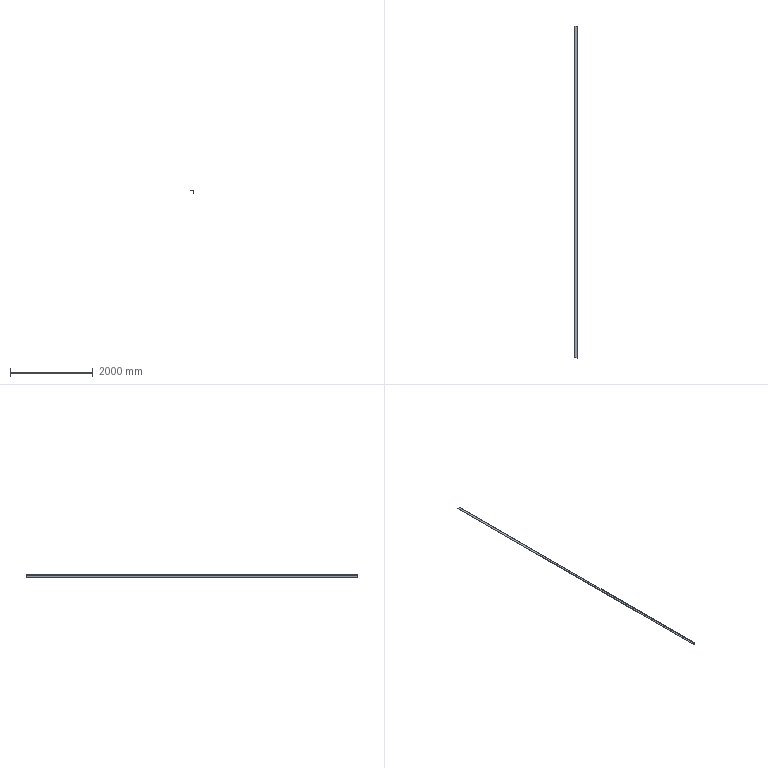Component | SolidWorks | 63#AngleIron-4 | 1 solid | 11 faces | box 63 x 8000 x 63 mm | volume 3982020 mm3 | plane 8 | cylinder 3 | commonest cylinder face diameters 2.667 x2 14 x1
build123d program:
from build123d import *

# Parameters (mm, degrees)
GB_T9787_1988_HOT_ROLLED_EQUAL_ANGLE_STE_DEPTH = 8000


with BuildPart() as part:
    # Sketch1 → Gb_t9787-1988 Hot Rolled Equal Angle Ste (new body)
    with BuildSketch(Plane.YZ):
        with BuildLine():
            Line((0, 0), (0, 63))
            Line((0, 63), (2.667, 63))
            ThreePointArc((2.667, 63), (3.609, 62.609), (4, 61.667))
            Line((4, 61.667), (4, 11))
            ThreePointArc((4, 11), (6.05, 6.05), (11, 4))
            Line((11, 4), (61.667, 4))
            ThreePointArc((61.667, 4), (62.609, 3.609), (63, 2.667))
            Line((63, 2.667), (63, 0))
            Line((63, 0), (0, 0))
        make_face()
    extrude(amount=GB_T9787_1988_HOT_ROLLED_EQUAL_ANGLE_STE_DEPTH)


solid = part.part

# Placed as in the assembly
solid = solid.moved(Location((2069.926, -31194.846, 4759), (-90, -90, 0)))
STEP:
#1=COLOUR_RGB('',0.7922,0.8196,0.9333);
#2=FILL_AREA_STYLE_COLOUR('',#1);
#3=FILL_AREA_STYLE('',(#2));
#4=SURFACE_STYLE_FILL_AREA(#3);
#5=SURFACE_SIDE_STYLE('',(#4));
#6=SURFACE_STYLE_USAGE(.BOTH.,#5);
#7=PRESENTATION_STYLE_ASSIGNMENT((#6));
#8=CARTESIAN_POINT('',(81.493,-1228.144,187.362));
#9=VERTEX_POINT('',#8);
#10=CARTESIAN_POINT('',(81.493,-1228.144,184.882));
#11=VERTEX_POINT('',#10);
#12=CARTESIAN_POINT('',(81.493,-1228.144,184.882));
#13=DIRECTION('',(-0.,-0.,-1.));
#14=VECTOR('',#13,39.37);
#15=LINE('',#12,#14);
#16=EDGE_CURVE('',#9,#11,#15,.T.);
#17=ORIENTED_EDGE('',*,*,#16,.T.);
#18=CARTESIAN_POINT('',(81.493,-913.183,184.882));
#19=VERTEX_POINT('',#18);
#20=CARTESIAN_POINT('',(81.493,-913.183,184.882));
#21=DIRECTION('',(-0.,-1.,0.));
#22=VECTOR('',#21,39.37);
#23=LINE('',#20,#22);
#24=EDGE_CURVE('',#19,#11,#23,.T.);
#25=ORIENTED_EDGE('',*,*,#24,.F.);
#26=CARTESIAN_POINT('',(81.493,-913.183,187.362));
#27=VERTEX_POINT('',#26);
#28=CARTESIAN_POINT('',(81.493,-913.183,184.882));
#29=DIRECTION('',(-0.,-0.,-1.));
#30=VECTOR('',#29,39.37);
#31=LINE('',#28,#30);
#32=EDGE_CURVE('',#27,#19,#31,.T.);
#33=ORIENTED_EDGE('',*,*,#32,.F.);
#34=CARTESIAN_POINT('',(81.493,-913.183,187.362));
#35=DIRECTION('',(-0.,-1.,0.));
#36=VECTOR('',#35,39.37);
#37=LINE('',#34,#36);
#38=EDGE_CURVE('',#27,#9,#37,.T.);
#39=ORIENTED_EDGE('',*,*,#38,.T.);
#40=EDGE_LOOP('',(#17,#25,#33,#39));
#41=FACE_OUTER_BOUND('',#40,.T.);
#42=CARTESIAN_POINT('',(81.493,-913.183,184.882));
#43=DIRECTION('',(-1.,0.,0.));
#44=DIRECTION('',(0.,1.,-0.));
#45=AXIS2_PLACEMENT_3D('',#42,#43,#44);
#46=PLANE('',#45);
#47=ADVANCED_FACE('',(#41),#46,.F.);
#48=CARTESIAN_POINT('',(81.388,-1228.144,184.882));
#49=VERTEX_POINT('',#48);
#50=CARTESIAN_POINT('',(81.493,-1228.144,184.882));
#51=DIRECTION('',(-1.,0.,0.));
#52=VECTOR('',#51,39.37);
#53=LINE('',#50,#52);
#54=EDGE_CURVE('',#11,#49,#53,.T.);
#55=ORIENTED_EDGE('',*,*,#54,.T.);
#56=CARTESIAN_POINT('',(81.388,-913.183,184.882));
#57=VERTEX_POINT('',#56);
#58=CARTESIAN_POINT('',(81.388,-913.183,184.882));
#59=DIRECTION('',(-0.,-1.,0.));
#60=VECTOR('',#59,39.37);
#61=LINE('',#58,#60);
#62=EDGE_CURVE('',#57,#49,#61,.T.);
#63=ORIENTED_EDGE('',*,*,#62,.F.);
#64=CARTESIAN_POINT('',(81.493,-913.183,184.882));
#65=DIRECTION('',(-1.,0.,0.));
#66=VECTOR('',#65,39.37);
#67=LINE('',#64,#66);
#68=EDGE_CURVE('',#19,#57,#67,.T.);
#69=ORIENTED_EDGE('',*,*,#68,.F.);
#70=ORIENTED_EDGE('',*,*,#24,.T.);
#71=EDGE_LOOP('',(#55,#63,#69,#70));
#72=FACE_OUTER_BOUND('',#71,.T.);
#73=CARTESIAN_POINT('',(81.493,-913.183,184.882));
#74=DIRECTION('',(0.,0.,1.));
#75=DIRECTION('',(1.,-0.,-0.));
#76=AXIS2_PLACEMENT_3D('',#73,#74,#75);
#77=PLANE('',#76);
#78=ADVANCED_FACE('',(#72),#77,.F.);
#79=CARTESIAN_POINT('',(81.336,-1228.144,184.934));
#80=VERTEX_POINT('',#79);
#81=CARTESIAN_POINT('',(81.388,-1228.144,184.934));
#82=DIRECTION('',(0.,1.,-0.));
#83=DIRECTION('',(1.,0.,0.));
#84=AXIS2_PLACEMENT_3D('',#81,#82,#83);
#85=CIRCLE('',#84,0.05249);
#86=EDGE_CURVE('',#49,#80,#85,.T.);
#87=ORIENTED_EDGE('',*,*,#86,.T.);
#88=CARTESIAN_POINT('',(81.336,-913.183,184.934));
#89=VERTEX_POINT('',#88);
#90=CARTESIAN_POINT('',(81.336,-913.183,184.934));
#91=DIRECTION('',(-0.,-1.,0.));
#92=VECTOR('',#91,39.37);
#93=LINE('',#90,#92);
#94=EDGE_CURVE('',#89,#80,#93,.T.);
#95=ORIENTED_EDGE('',*,*,#94,.F.);
#96=CARTESIAN_POINT('',(81.388,-913.183,184.934));
#97=DIRECTION('',(0.,1.,-0.));
#98=DIRECTION('',(1.,0.,0.));
#99=AXIS2_PLACEMENT_3D('',#96,#97,#98);
#100=CIRCLE('',#99,0.05249);
#101=EDGE_CURVE('',#57,#89,#100,.T.);
#102=ORIENTED_EDGE('',*,*,#101,.F.);
#103=ORIENTED_EDGE('',*,*,#62,.T.);
#104=EDGE_LOOP('',(#87,#95,#102,#103));
#105=FACE_OUTER_BOUND('',#104,.T.);
#106=CARTESIAN_POINT('',(81.388,-913.183,184.934));
#107=DIRECTION('',(-0.,-1.,0.));
#108=DIRECTION('',(-1.,0.,0.));
#109=AXIS2_PLACEMENT_3D('',#106,#107,#108);
#110=CYLINDRICAL_SURFACE('',#109,0.05249);
#111=ADVANCED_FACE('',(#105),#110,.T.);
#112=CARTESIAN_POINT('',(81.336,-1228.144,186.929));
#113=VERTEX_POINT('',#112);
#114=CARTESIAN_POINT('',(81.336,-1228.144,186.929));
#115=DIRECTION('',(0.,0.,1.));
#116=VECTOR('',#115,39.37);
#117=LINE('',#114,#116);
#118=EDGE_CURVE('',#80,#113,#117,.T.);
#119=ORIENTED_EDGE('',*,*,#118,.T.);
#120=CARTESIAN_POINT('',(81.336,-913.183,186.929));
#121=VERTEX_POINT('',#120);
#122=CARTESIAN_POINT('',(81.336,-913.183,186.929));
#123=DIRECTION('',(-0.,-1.,0.));
#124=VECTOR('',#123,39.37);
#125=LINE('',#122,#124);
#126=EDGE_CURVE('',#121,#113,#125,.T.);
#127=ORIENTED_EDGE('',*,*,#126,.F.);
#128=CARTESIAN_POINT('',(81.336,-913.183,186.929));
#129=DIRECTION('',(0.,0.,1.));
#130=VECTOR('',#129,39.37);
#131=LINE('',#128,#130);
#132=EDGE_CURVE('',#89,#121,#131,.T.);
#133=ORIENTED_EDGE('',*,*,#132,.F.);
#134=ORIENTED_EDGE('',*,*,#94,.T.);
#135=EDGE_LOOP('',(#119,#127,#133,#134));
#136=FACE_OUTER_BOUND('',#135,.T.);
#137=CARTESIAN_POINT('',(81.336,-913.183,186.929));
#138=DIRECTION('',(1.,-0.,-0.));
#139=DIRECTION('',(-0.,-0.,-1.));
#140=AXIS2_PLACEMENT_3D('',#137,#138,#139);
#141=PLANE('',#140);
#142=ADVANCED_FACE('',(#136),#141,.F.);
#143=CARTESIAN_POINT('',(81.06,-1228.144,187.205));
#144=VERTEX_POINT('',#143);
#145=CARTESIAN_POINT('',(81.06,-1228.144,186.929));
#146=DIRECTION('',(-0.,-1.,0.));
#147=DIRECTION('',(-1.,0.,0.));
#148=AXIS2_PLACEMENT_3D('',#145,#146,#147);
#149=CIRCLE('',#148,0.2756);
#150=EDGE_CURVE('',#113,#144,#149,.T.);
#151=ORIENTED_EDGE('',*,*,#150,.T.);
#152=CARTESIAN_POINT('',(81.06,-913.183,187.205));
#153=VERTEX_POINT('',#152);
#154=CARTESIAN_POINT('',(81.06,-913.183,187.205));
#155=DIRECTION('',(-0.,-1.,0.));
#156=VECTOR('',#155,39.37);
#157=LINE('',#154,#156);
#158=EDGE_CURVE('',#153,#144,#157,.T.);
#159=ORIENTED_EDGE('',*,*,#158,.F.);
#160=CARTESIAN_POINT('',(81.06,-913.183,186.929));
#161=DIRECTION('',(-0.,-1.,0.));
#162=DIRECTION('',(-1.,0.,0.));
#163=AXIS2_PLACEMENT_3D('',#160,#161,#162);
#164=CIRCLE('',#163,0.2756);
#165=EDGE_CURVE('',#121,#153,#164,.T.);
#166=ORIENTED_EDGE('',*,*,#165,.F.);
#167=ORIENTED_EDGE('',*,*,#126,.T.);
#168=EDGE_LOOP('',(#151,#159,#166,#167));
#169=FACE_OUTER_BOUND('',#168,.T.);
#170=CARTESIAN_POINT('',(81.06,-913.183,186.929));
#171=DIRECTION('',(-0.,-1.,0.));
#172=DIRECTION('',(-1.,0.,0.));
#173=AXIS2_PLACEMENT_3D('',#170,#171,#172);
#174=CYLINDRICAL_SURFACE('',#173,0.2756);
#175=ADVANCED_FACE('',(#169),#174,.F.);
#176=CARTESIAN_POINT('',(79.065,-1228.144,187.205));
#177=VERTEX_POINT('',#176);
#178=CARTESIAN_POINT('',(79.065,-1228.144,187.205));
#179=DIRECTION('',(-1.,0.,0.));
#180=VECTOR('',#179,39.37);
#181=LINE('',#178,#180);
#182=EDGE_CURVE('',#144,#177,#181,.T.);
#183=ORIENTED_EDGE('',*,*,#182,.T.);
#184=CARTESIAN_POINT('',(79.065,-913.183,187.205));
#185=VERTEX_POINT('',#184);
#186=CARTESIAN_POINT('',(79.065,-913.183,187.205));
#187=DIRECTION('',(-0.,-1.,0.));
#188=VECTOR('',#187,39.37);
#189=LINE('',#186,#188);
#190=EDGE_CURVE('',#185,#177,#189,.T.);
#191=ORIENTED_EDGE('',*,*,#190,.F.);
#192=CARTESIAN_POINT('',(79.065,-913.183,187.205));
#193=DIRECTION('',(-1.,0.,0.));
#194=VECTOR('',#193,39.37);
#195=LINE('',#192,#194);
#196=EDGE_CURVE('',#153,#185,#195,.T.);
#197=ORIENTED_EDGE('',*,*,#196,.F.);
#198=ORIENTED_EDGE('',*,*,#158,.T.);
#199=EDGE_LOOP('',(#183,#191,#197,#198));
#200=FACE_OUTER_BOUND('',#199,.T.);
#201=CARTESIAN_POINT('',(79.065,-913.183,187.205));
#202=DIRECTION('',(0.,0.,1.));
#203=DIRECTION('',(1.,-0.,-0.));
#204=AXIS2_PLACEMENT_3D('',#201,#202,#203);
#205=PLANE('',#204);
#206=ADVANCED_FACE('',(#200),#205,.F.);
#207=CARTESIAN_POINT('',(79.013,-1228.144,187.257));
#208=VERTEX_POINT('',#207);
#209=CARTESIAN_POINT('',(79.065,-1228.144,187.257));
#210=DIRECTION('',(0.,1.,-0.));
#211=DIRECTION('',(-1.,0.,0.));
#212=AXIS2_PLACEMENT_3D('',#209,#210,#211);
#213=CIRCLE('',#212,0.05249);
#214=EDGE_CURVE('',#177,#208,#213,.T.);
#215=ORIENTED_EDGE('',*,*,#214,.T.);
#216=CARTESIAN_POINT('',(79.013,-913.183,187.257));
#217=VERTEX_POINT('',#216);
#218=CARTESIAN_POINT('',(79.013,-913.183,187.257));
#219=DIRECTION('',(-0.,-1.,0.));
#220=VECTOR('',#219,39.37);
#221=LINE('',#218,#220);
#222=EDGE_CURVE('',#217,#208,#221,.T.);
#223=ORIENTED_EDGE('',*,*,#222,.F.);
#224=CARTESIAN_POINT('',(79.065,-913.183,187.257));
#225=DIRECTION('',(0.,1.,-0.));
#226=DIRECTION('',(-1.,0.,0.));
#227=AXIS2_PLACEMENT_3D('',#224,#225,#226);
#228=CIRCLE('',#227,0.05249);
#229=EDGE_CURVE('',#185,#217,#228,.T.);
#230=ORIENTED_EDGE('',*,*,#229,.F.);
#231=ORIENTED_EDGE('',*,*,#190,.T.);
#232=EDGE_LOOP('',(#215,#223,#230,#231));
#233=FACE_OUTER_BOUND('',#232,.T.);
#234=CARTESIAN_POINT('',(79.065,-913.183,187.257));
#235=DIRECTION('',(-0.,-1.,0.));
#236=DIRECTION('',(-1.,0.,0.));
#237=AXIS2_PLACEMENT_3D('',#234,#235,#236);
#238=CYLINDRICAL_SURFACE('',#237,0.05249);
#239=ADVANCED_FACE('',(#233),#238,.T.);
#240=CARTESIAN_POINT('',(79.013,-1228.144,187.362));
#241=VERTEX_POINT('',#240);
#242=CARTESIAN_POINT('',(79.013,-1228.144,187.362));
#243=DIRECTION('',(0.,0.,1.));
#244=VECTOR('',#243,39.37);
#245=LINE('',#242,#244);
#246=EDGE_CURVE('',#208,#241,#245,.T.);
#247=ORIENTED_EDGE('',*,*,#246,.T.);
#248=CARTESIAN_POINT('',(79.013,-913.183,187.362));
#249=VERTEX_POINT('',#248);
#250=CARTESIAN_POINT('',(79.013,-913.183,187.362));
#251=DIRECTION('',(-0.,-1.,0.));
#252=VECTOR('',#251,39.37);
#253=LINE('',#250,#252);
#254=EDGE_CURVE('',#249,#241,#253,.T.);
#255=ORIENTED_EDGE('',*,*,#254,.F.);
#256=CARTESIAN_POINT('',(79.013,-913.183,187.362));
#257=DIRECTION('',(0.,0.,1.));
#258=VECTOR('',#257,39.37);
#259=LINE('',#256,#258);
#260=EDGE_CURVE('',#217,#249,#259,.T.);
#261=ORIENTED_EDGE('',*,*,#260,.F.);
#262=ORIENTED_EDGE('',*,*,#222,.T.);
#263=EDGE_LOOP('',(#247,#255,#261,#262));
#264=FACE_OUTER_BOUND('',#263,.T.);
#265=CARTESIAN_POINT('',(79.013,-913.183,187.362));
#266=DIRECTION('',(1.,-0.,-0.));
#267=DIRECTION('',(-0.,-1.,0.));
#268=AXIS2_PLACEMENT_3D('',#265,#266,#267);
#269=PLANE('',#268);
#270=ADVANCED_FACE('',(#264),#269,.F.);
#271=CARTESIAN_POINT('',(81.493,-1228.144,187.362));
#272=DIRECTION('',(1.,-0.,-0.));
#273=VECTOR('',#272,39.37);
#274=LINE('',#271,#273);
#275=EDGE_CURVE('',#241,#9,#274,.T.);
#276=ORIENTED_EDGE('',*,*,#275,.T.);
#277=ORIENTED_EDGE('',*,*,#38,.F.);
#278=CARTESIAN_POINT('',(81.493,-913.183,187.362));
#279=DIRECTION('',(1.,-0.,-0.));
#280=VECTOR('',#279,39.37);
#281=LINE('',#278,#280);
#282=EDGE_CURVE('',#249,#27,#281,.T.);
#283=ORIENTED_EDGE('',*,*,#282,.F.);
#284=ORIENTED_EDGE('',*,*,#254,.T.);
#285=EDGE_LOOP('',(#276,#277,#283,#284));
#286=FACE_OUTER_BOUND('',#285,.T.);
#287=CARTESIAN_POINT('',(81.493,-913.183,187.362));
#288=DIRECTION('',(-0.,-0.,-1.));
#289=DIRECTION('',(-1.,0.,0.));
#290=AXIS2_PLACEMENT_3D('',#287,#288,#289);
#291=PLANE('',#290);
#292=ADVANCED_FACE('',(#286),#291,.F.);
#293=ORIENTED_EDGE('',*,*,#32,.T.);
#294=ORIENTED_EDGE('',*,*,#68,.T.);
#295=ORIENTED_EDGE('',*,*,#101,.T.);
#296=ORIENTED_EDGE('',*,*,#132,.T.);
#297=ORIENTED_EDGE('',*,*,#165,.T.);
#298=ORIENTED_EDGE('',*,*,#196,.T.);
#299=ORIENTED_EDGE('',*,*,#229,.T.);
#300=ORIENTED_EDGE('',*,*,#260,.T.);
#301=ORIENTED_EDGE('',*,*,#282,.T.);
#302=EDGE_LOOP('',(#293,#294,#295,#296,#297,#298,#299,#300,#301));
#303=FACE_OUTER_BOUND('',#302,.T.);
#304=CARTESIAN_POINT('',(79.065,-913.183,187.257));
#305=DIRECTION('',(-0.,-1.,0.));
#306=DIRECTION('',(-1.,0.,0.));
#307=AXIS2_PLACEMENT_3D('',#304,#305,#306);
#308=PLANE('',#307);
#309=ADVANCED_FACE('',(#303),#308,.F.);
#310=ORIENTED_EDGE('',*,*,#16,.F.);
#311=ORIENTED_EDGE('',*,*,#275,.F.);
#312=ORIENTED_EDGE('',*,*,#246,.F.);
#313=ORIENTED_EDGE('',*,*,#214,.F.);
#314=ORIENTED_EDGE('',*,*,#182,.F.);
#315=ORIENTED_EDGE('',*,*,#150,.F.);
#316=ORIENTED_EDGE('',*,*,#118,.F.);
#317=ORIENTED_EDGE('',*,*,#86,.F.);
#318=ORIENTED_EDGE('',*,*,#54,.F.);
#319=EDGE_LOOP('',(#310,#311,#312,#313,#314,#315,#316,#317,#318));
#320=FACE_OUTER_BOUND('',#319,.T.);
#321=CARTESIAN_POINT('',(79.065,-1228.144,187.257));
#322=DIRECTION('',(-0.,-1.,0.));
#323=DIRECTION('',(-1.,0.,0.));
#324=AXIS2_PLACEMENT_3D('',#321,#322,#323);
#325=PLANE('',#324);
#326=ADVANCED_FACE('',(#320),#325,.T.);
#327=CLOSED_SHELL('',(#47,#78,#111,#142,#175,#206,#239,#270,#292,#309,#326));
#328=MANIFOLD_SOLID_BREP('',#327);
#329=STYLED_ITEM('',(#7),#328);
#330=(LENGTH_UNIT()NAMED_UNIT(*)SI_UNIT($,.METRE.));
#331=LENGTH_MEASURE_WITH_UNIT(LENGTH_MEASURE(0.0254),#330);
#332=DIMENSIONAL_EXPONENTS(1.,0.,0.,0.,0.,0.,0.);
#333=(CONVERSION_BASED_UNIT('',#331)LENGTH_UNIT()NAMED_UNIT(#332));
#334=UNCERTAINTY_MEASURE_WITH_UNIT(LENGTH_MEASURE(0.00001),#333,'','');
#335=(NAMED_UNIT(*)PLANE_ANGLE_UNIT()SI_UNIT($,.RADIAN.));
#336=(NAMED_UNIT(*)SI_UNIT($,.STERADIAN.)SOLID_ANGLE_UNIT());
#337=(GEOMETRIC_REPRESENTATION_CONTEXT(3)GLOBAL_UNCERTAINTY_ASSIGNED_CONTEXT((#334))GLOBAL_UNIT_ASSIGNED_CONTEXT((#333,#335,#336))REPRESENTATION_CONTEXT('',''));
#338=MECHANICAL_DESIGN_GEOMETRIC_PRESENTATION_REPRESENTATION('',(#329),#337);
#339=CARTESIAN_POINT('',(0.,0.,0.));
#340=DIRECTION('',(0.,0.,1.));
#341=DIRECTION('',(1.,0.,0.));
#342=AXIS2_PLACEMENT_3D('',#339,#340,#341);
#343=(LENGTH_UNIT()NAMED_UNIT(*)SI_UNIT($,.METRE.));
#344=LENGTH_MEASURE_WITH_UNIT(LENGTH_MEASURE(0.0254),#343);
#345=DIMENSIONAL_EXPONENTS(1.,0.,0.,0.,0.,0.,0.);
#346=(CONVERSION_BASED_UNIT('',#344)LENGTH_UNIT()NAMED_UNIT(#345));
#347=UNCERTAINTY_MEASURE_WITH_UNIT(LENGTH_MEASURE(0.00001),#346,'','');
#348=(NAMED_UNIT(*)PLANE_ANGLE_UNIT()SI_UNIT($,.RADIAN.));
#349=(NAMED_UNIT(*)SI_UNIT($,.STERADIAN.)SOLID_ANGLE_UNIT());
#350=(GEOMETRIC_REPRESENTATION_CONTEXT(3)GLOBAL_UNCERTAINTY_ASSIGNED_CONTEXT((#347))GLOBAL_UNIT_ASSIGNED_CONTEXT((#346,#348,#349))REPRESENTATION_CONTEXT('',''));
#351=ADVANCED_BREP_SHAPE_REPRESENTATION('',(#328,#342),#350);
#352=PRESENTATION_LAYER_ASSIGNMENT('','',(#329));